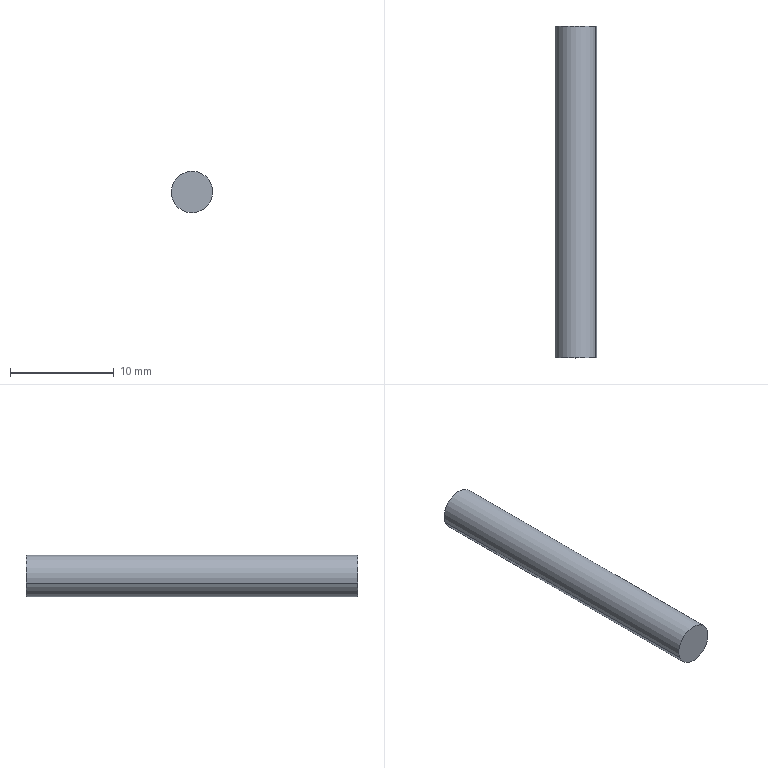Component | SolidWorks | OpticalAxis_4_32-1 | 1 solid | 4 faces | box 4 x 32 x 4 mm | volume 402 mm3 | cylinder 2 | plane 2 | commonest cylinder face diameters 4 x2 | material Q235-A
build123d program:
from build123d import *

# Parameters (mm, degrees)
SKETCH1_R      = 2
EXTRUDE1_DEPTH = 16


with BuildPart() as part:
    # Sketch1 → Extrude1 (new, symmetric)
    with BuildSketch(Plane.XY):
        Circle(SKETCH1_R)
    extrude(amount=EXTRUDE1_DEPTH, both=True)


solid = part.part

# Placed as in the assembly
solid = solid.moved(Location((210.87, 43.668, 34.729), (90, 0, 0)))
STEP:
#1=COLOUR_RGB('',0.7922,0.8196,0.9333);
#2=FILL_AREA_STYLE_COLOUR('',#1);
#3=FILL_AREA_STYLE('',(#2));
#4=SURFACE_STYLE_FILL_AREA(#3);
#5=SURFACE_SIDE_STYLE('',(#4));
#6=SURFACE_STYLE_USAGE(.BOTH.,#5);
#7=PRESENTATION_STYLE_ASSIGNMENT((#6));
#8=CARTESIAN_POINT('',(8.376,1.089,1.394));
#9=VERTEX_POINT('',#8);
#10=CARTESIAN_POINT('',(8.228,1.089,1.341));
#11=VERTEX_POINT('',#10);
#12=CARTESIAN_POINT('',(8.302,1.089,1.367));
#13=DIRECTION('',(0.,-1.,-0.));
#14=DIRECTION('',(0.941,0.,0.3384));
#15=AXIS2_PLACEMENT_3D('',#12,#13,#14);
#16=CIRCLE('',#15,0.07874);
#17=EDGE_CURVE('',#9,#11,#16,.T.);
#18=ORIENTED_EDGE('',*,*,#17,.F.);
#19=CARTESIAN_POINT('',(8.376,2.349,1.394));
#20=VERTEX_POINT('',#19);
#21=CARTESIAN_POINT('',(8.376,1.089,1.394));
#22=DIRECTION('',(-0.,1.,0.));
#23=VECTOR('',#22,39.37);
#24=LINE('',#21,#23);
#25=EDGE_CURVE('',#9,#20,#24,.T.);
#26=ORIENTED_EDGE('',*,*,#25,.T.);
#27=CARTESIAN_POINT('',(8.228,2.349,1.341));
#28=VERTEX_POINT('',#27);
#29=CARTESIAN_POINT('',(8.302,2.349,1.367));
#30=DIRECTION('',(0.,-1.,-0.));
#31=DIRECTION('',(0.941,0.,0.3384));
#32=AXIS2_PLACEMENT_3D('',#29,#30,#31);
#33=CIRCLE('',#32,0.07874);
#34=EDGE_CURVE('',#20,#28,#33,.T.);
#35=ORIENTED_EDGE('',*,*,#34,.T.);
#36=CARTESIAN_POINT('',(8.228,1.089,1.341));
#37=DIRECTION('',(-0.,1.,0.));
#38=VECTOR('',#37,39.37);
#39=LINE('',#36,#38);
#40=EDGE_CURVE('',#11,#28,#39,.T.);
#41=ORIENTED_EDGE('',*,*,#40,.F.);
#42=EDGE_LOOP('',(#18,#26,#35,#41));
#43=FACE_OUTER_BOUND('',#42,.T.);
#44=CARTESIAN_POINT('',(8.302,1.089,1.367));
#45=DIRECTION('',(-0.,1.,0.));
#46=DIRECTION('',(-0.941,0.,-0.3384));
#47=AXIS2_PLACEMENT_3D('',#44,#45,#46);
#48=CYLINDRICAL_SURFACE('',#47,0.07874);
#49=ADVANCED_FACE('',(#43),#48,.T.);
#50=ORIENTED_EDGE('',*,*,#25,.F.);
#51=CARTESIAN_POINT('',(8.302,1.089,1.367));
#52=DIRECTION('',(0.,-1.,-0.));
#53=DIRECTION('',(0.941,0.,0.3384));
#54=AXIS2_PLACEMENT_3D('',#51,#52,#53);
#55=CIRCLE('',#54,0.07874);
#56=EDGE_CURVE('',#11,#9,#55,.T.);
#57=ORIENTED_EDGE('',*,*,#56,.F.);
#58=ORIENTED_EDGE('',*,*,#40,.T.);
#59=CARTESIAN_POINT('',(8.302,2.349,1.367));
#60=DIRECTION('',(0.,-1.,-0.));
#61=DIRECTION('',(0.941,0.,0.3384));
#62=AXIS2_PLACEMENT_3D('',#59,#60,#61);
#63=CIRCLE('',#62,0.07874);
#64=EDGE_CURVE('',#28,#20,#63,.T.);
#65=ORIENTED_EDGE('',*,*,#64,.T.);
#66=EDGE_LOOP('',(#50,#57,#58,#65));
#67=FACE_OUTER_BOUND('',#66,.T.);
#68=CARTESIAN_POINT('',(8.302,1.089,1.367));
#69=DIRECTION('',(-0.,1.,0.));
#70=DIRECTION('',(-0.941,0.,-0.3384));
#71=AXIS2_PLACEMENT_3D('',#68,#69,#70);
#72=CYLINDRICAL_SURFACE('',#71,0.07874);
#73=ADVANCED_FACE('',(#67),#72,.T.);
#74=ORIENTED_EDGE('',*,*,#56,.T.);
#75=ORIENTED_EDGE('',*,*,#17,.T.);
#76=EDGE_LOOP('',(#74,#75));
#77=FACE_OUTER_BOUND('',#76,.T.);
#78=CARTESIAN_POINT('',(8.302,1.089,1.367));
#79=DIRECTION('',(0.,-1.,-0.));
#80=DIRECTION('',(0.941,0.,0.3384));
#81=AXIS2_PLACEMENT_3D('',#78,#79,#80);
#82=PLANE('',#81);
#83=ADVANCED_FACE('',(#77),#82,.T.);
#84=ORIENTED_EDGE('',*,*,#64,.F.);
#85=ORIENTED_EDGE('',*,*,#34,.F.);
#86=EDGE_LOOP('',(#84,#85));
#87=FACE_OUTER_BOUND('',#86,.T.);
#88=CARTESIAN_POINT('',(8.302,2.349,1.367));
#89=DIRECTION('',(0.,-1.,-0.));
#90=DIRECTION('',(0.941,0.,0.3384));
#91=AXIS2_PLACEMENT_3D('',#88,#89,#90);
#92=PLANE('',#91);
#93=ADVANCED_FACE('',(#87),#92,.F.);
#94=CLOSED_SHELL('',(#49,#73,#83,#93));
#95=MANIFOLD_SOLID_BREP('',#94);
#96=STYLED_ITEM('',(#7),#95);
#97=PRESENTATION_LAYER_ASSIGNMENT('','',(#96));
#98=(LENGTH_UNIT()NAMED_UNIT(*)SI_UNIT($,.METRE.));
#99=LENGTH_MEASURE_WITH_UNIT(LENGTH_MEASURE(0.0254),#98);
#100=DIMENSIONAL_EXPONENTS(1.,0.,0.,0.,0.,0.,0.);
#101=(CONVERSION_BASED_UNIT('',#99)LENGTH_UNIT()NAMED_UNIT(#100));
#102=UNCERTAINTY_MEASURE_WITH_UNIT(LENGTH_MEASURE(0.00001),#101,'','');
#103=(NAMED_UNIT(*)PLANE_ANGLE_UNIT()SI_UNIT($,.RADIAN.));
#104=(NAMED_UNIT(*)SI_UNIT($,.STERADIAN.)SOLID_ANGLE_UNIT());
#105=(GEOMETRIC_REPRESENTATION_CONTEXT(3)GLOBAL_UNCERTAINTY_ASSIGNED_CONTEXT((#102))GLOBAL_UNIT_ASSIGNED_CONTEXT((#101,#103,#104))REPRESENTATION_CONTEXT('',''));
#106=MECHANICAL_DESIGN_GEOMETRIC_PRESENTATION_REPRESENTATION('',(#96),#105);
#107=CARTESIAN_POINT('',(0.,0.,0.));
#108=DIRECTION('',(0.,0.,1.));
#109=DIRECTION('',(1.,0.,0.));
#110=AXIS2_PLACEMENT_3D('',#107,#108,#109);
#111=(LENGTH_UNIT()NAMED_UNIT(*)SI_UNIT($,.METRE.));
#112=LENGTH_MEASURE_WITH_UNIT(LENGTH_MEASURE(0.0254),#111);
#113=DIMENSIONAL_EXPONENTS(1.,0.,0.,0.,0.,0.,0.);
#114=(CONVERSION_BASED_UNIT('',#112)LENGTH_UNIT()NAMED_UNIT(#113));
#115=UNCERTAINTY_MEASURE_WITH_UNIT(LENGTH_MEASURE(0.00001),#114,'','');
#116=(NAMED_UNIT(*)PLANE_ANGLE_UNIT()SI_UNIT($,.RADIAN.));
#117=(NAMED_UNIT(*)SI_UNIT($,.STERADIAN.)SOLID_ANGLE_UNIT());
#118=(GEOMETRIC_REPRESENTATION_CONTEXT(3)GLOBAL_UNCERTAINTY_ASSIGNED_CONTEXT((#115))GLOBAL_UNIT_ASSIGNED_CONTEXT((#114,#116,#117))REPRESENTATION_CONTEXT('',''));
#119=ADVANCED_BREP_SHAPE_REPRESENTATION('',(#95,#110),#118);